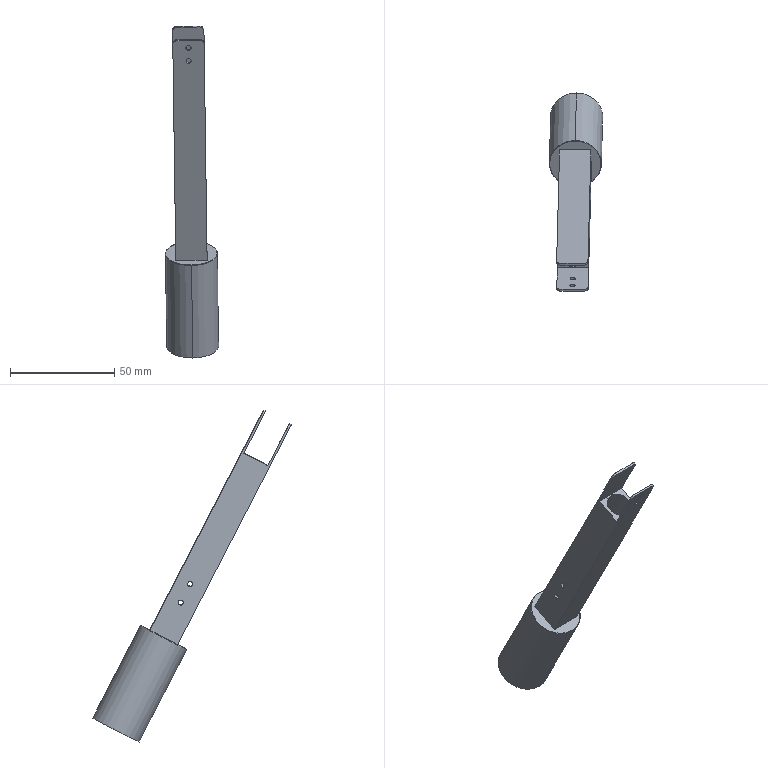Component | SolidWorks | 2018SOLIDWORKS1400000010-1 | 1 solid | 36 faces | box 25.61 x 95.11 x 158.94 mm | volume 26727 mm3 | cylinder 22 | plane 12 | cone 2 | commonest cylinder face diameters 2.5 x12 4 x4 18 x2 25 x2 12 x2 | material 45 Steel
build123d program:
from build123d import *

# Parameters (mm, degrees)
SKETCH1_R             = 12.5
BOSS_EXTRUDE1_DEPTH   = 50
SKETCH3_W             = 15
SKETCH3_H             = 15
BOSS_EXTRUDE2_DEPTH   = 120
SKETCH6_W             = 13
SKETCH6_H             = 24
CUT_EXTRUDE3_DEPTH    = 30
SKETCH7_R             = 6
CUT_EXTRUDE4_DEPTH    = 150
SKETCH8_R             = 9
CUT_EXTRUDE5_DEPTH    = 25
CHAMFER2_SIZE         = 0.2
SKETCH15_W            = 1
SKETCH15_H            = 15
BOSS_EXTRUDE3_DEPTH   = 2.5
SKETCH16_W            = 1
SKETCH16_H            = 15
CUT_EXTRUDE7_DEPTH    = 1.5
SKETCH18_W            = 4
SKETCH18_H            = 15
CUT_EXTRUDE8_DEPTH    = 125.593
M3_TAPPED_HOLE3_D     = 2.5
M3_TAPPED_HOLE3_DEPTH = 8.5
M3_TAPPED_HOLE3_TIP   = 0.7511
FILLET1_R             = 2
M3_TAPPED_HOLE4_D     = 2.5


with BuildPart() as part:
    # Sketch1 → Boss-Extrude1 (new body)
    with BuildSketch(Plane.XY):
        Circle(SKETCH1_R)
    extrude(amount=BOSS_EXTRUDE1_DEPTH)

    # Sketch3 → Boss-Extrude2 (add)
    with BuildSketch(Plane(origin=(0, 0, 0), x_dir=(-1, 0, 0), z_dir=(0, 0, -1))):
        Rectangle(SKETCH3_W, SKETCH3_H)
    extrude(amount=BOSS_EXTRUDE2_DEPTH)

    # Sketch6 → Cut-Extrude3 (cut)
    with BuildSketch(Plane.XZ.offset(7.5)):
        with Locations((0, -108)):
            Rectangle(SKETCH6_W, SKETCH6_H)
    extrude(amount=-CUT_EXTRUDE3_DEPTH, mode=Mode.SUBTRACT)

    # Sketch7 → Cut-Extrude4 (cut)
    with BuildSketch(Plane.XY.offset(50)):
        Circle(SKETCH7_R)
    extrude(amount=-CUT_EXTRUDE4_DEPTH, mode=Mode.SUBTRACT)

    # Sketch8 → Cut-Extrude5 (cut)
    with BuildSketch(Plane.XY.offset(50)):
        Circle(SKETCH8_R)
    extrude(amount=-CUT_EXTRUDE5_DEPTH, mode=Mode.SUBTRACT)

    # Chamfer2
    chamfer2_edges = [part.edges().sort_by_distance(p)[0] for p in [
        (-12.5, 0, 0),
    ]]
    chamfer(chamfer2_edges, length=CHAMFER2_SIZE)

    # Sketch15 → Boss-Extrude3 (add)
    with BuildSketch(Plane(origin=(0, 0, -120), x_dir=(-1, 0, 0), z_dir=(0, 0, -1))):
        with Locations((-7, 0)):
            Rectangle(SKETCH15_W, SKETCH15_H)
    extrude(amount=BOSS_EXTRUDE3_DEPTH)

    # Sketch16 → Cut-Extrude7 (cut)
    with BuildSketch(Plane(origin=(0, 0, -120), x_dir=(-1, 0, 0), z_dir=(0, 0, -1))):
        with Locations((7, 0)):
            Rectangle(SKETCH16_W, SKETCH16_H)
    extrude(amount=-CUT_EXTRUDE7_DEPTH, mode=Mode.SUBTRACT)

    # Sketch18 → Cut-Extrude8 (cut, through all)
    with BuildSketch(Plane.ZY.offset(-6.5)):
        with Locations((-120.5, 0)):
            Rectangle(SKETCH18_W, SKETCH18_H)
    extrude(amount=-CUT_EXTRUDE8_DEPTH, mode=Mode.SUBTRACT)

    # M3 Tapped Hole3
    with Locations(Plane(origin=(7.5, 0, 0), x_dir=(0, 0, -1), z_dir=(1, 0, 0))):
        with Locations((114.5, 0), (107.5, 0)):
            Hole(M3_TAPPED_HOLE3_D / 2, depth=M3_TAPPED_HOLE3_DEPTH)
            with Locations((0, 0, -(M3_TAPPED_HOLE3_DEPTH + M3_TAPPED_HOLE3_TIP / 2))):  # 118° drill point
                Cone(0, M3_TAPPED_HOLE3_D / 2, M3_TAPPED_HOLE3_TIP, mode=Mode.SUBTRACT)

    # Fillet1
    fillet1_edges = [part.edges().sort_by_distance(p)[0] for p in [
        (-7, 7.5, -118.5),
        (-7, -7.5, -118.5),
        (7, 7.5, -118.5),
        (7, -7.5, -118.5),
    ]]
    fillet(fillet1_edges, radius=FILLET1_R)

    # M3 Tapped Hole4 (through all)
    with Locations(Plane(origin=(0, 7.5, 0), x_dir=(1, 0, 0), z_dir=(0, 1, 0))):
        with Locations((-0.5, 28.5), (-0.5, 18.5)):
            Hole(M3_TAPPED_HOLE4_D / 2)


solid = part.part

# Placed as in the assembly
solid = solid.moved(Location((97.894, -54.442, 91.514), (-152.675, 0.7042, 89.636)))